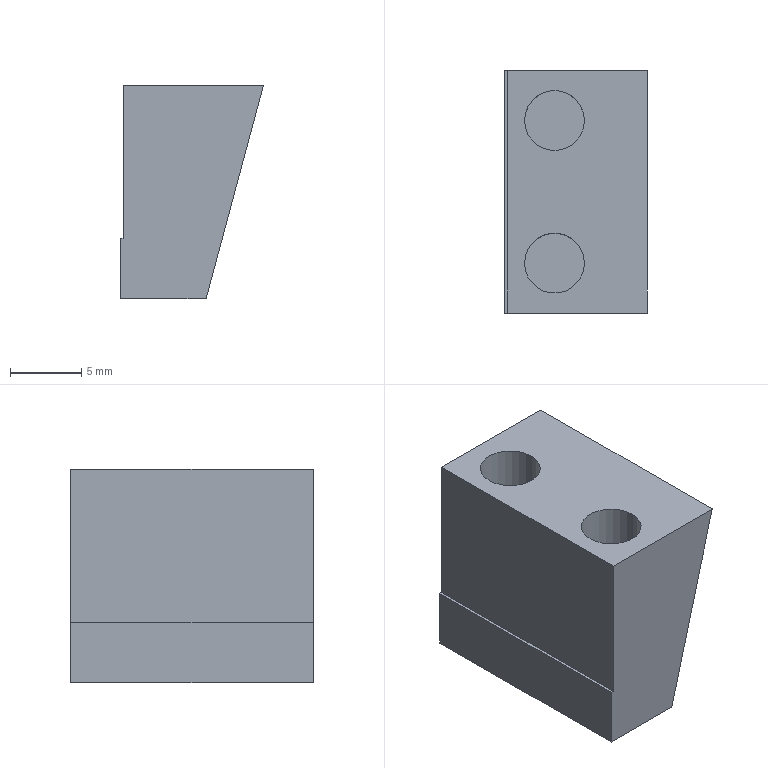Component | SolidWorks | 8TC-A15004-60-31A-4 | 1 solid | 14 faces | box 10.02 x 17 x 15 mm | volume 1770 mm3 | plane 10 | cylinder 4 | commonest cylinder face diameters 4.2 x4 | material #45
build123d program:
from build123d import *

# Parameters (mm, degrees)
BOSS_EXTRUDE1_DEPTH      = 8.5
M4_CLEARANCE_HOLE1_D     = 4.2
M4_CLEARANCE_HOLE1_DEPTH = 8.5
SKETCH1_W                = 0.7
SKETCH1_H                = 11.25
BLADESEATRELIEF_DEPTH    = 15


with BuildPart() as part:
    # Sketch1_2 → Boss-Extrude1 (new, symmetric)
    with BuildSketch(Plane(origin=(0, 0, 0), x_dir=(1, 0, 0), z_dir=(0, 1, 0))):
        Polygon((-7.019, 0), (3, 0), (3, 15), (-3, 15), align=None)
    extrude(amount=BOSS_EXTRUDE1_DEPTH, both=True)

    # M4 Clearance Hole1
    with Locations(Plane.XY):
        with Locations((-0.5, 5), (-0.5, -5)):
            Hole(M4_CLEARANCE_HOLE1_D / 2, depth=M4_CLEARANCE_HOLE1_DEPTH)

    # Sketch1 → BladeSeatRelief (cut, symmetric)
    with BuildSketch(Plane(origin=(0, 0, 0), x_dir=(1, 0, 0), z_dir=(0, 1, 0))):
        with Locations((3.15, 5.125)):
            Rectangle(SKETCH1_W, SKETCH1_H)
    extrude(amount=BLADESEATRELIEF_DEPTH, both=True, mode=Mode.SUBTRACT)


solid = part.part

# Placed as in the assembly
solid = solid.moved(Location((47.714, -68.5, 6), (0, 0, 180)))
STEP:
#1=COLOUR_RGB('',0.7922,0.8196,0.9333);
#2=FILL_AREA_STYLE_COLOUR('',#1);
#3=FILL_AREA_STYLE('',(#2));
#4=SURFACE_STYLE_FILL_AREA(#3);
#5=SURFACE_SIDE_STYLE('',(#4));
#6=SURFACE_STYLE_USAGE(.BOTH.,#5);
#7=PRESENTATION_STYLE_ASSIGNMENT((#6));
#8=CARTESIAN_POINT('',(1.981,-2.894,-0.09843));
#9=VERTEX_POINT('',#8);
#10=CARTESIAN_POINT('',(1.816,-2.894,-0.09843));
#11=VERTEX_POINT('',#10);
#12=CARTESIAN_POINT('',(1.898,-2.894,-0.09843));
#13=DIRECTION('',(0.,-0.,1.));
#14=DIRECTION('',(-1.,0.,0.));
#15=AXIS2_PLACEMENT_3D('',#12,#13,#14);
#16=CIRCLE('',#15,0.08268);
#17=EDGE_CURVE('',#9,#11,#16,.T.);
#18=ORIENTED_EDGE('',*,*,#17,.F.);
#19=CARTESIAN_POINT('',(1.981,-2.894,0.2362));
#20=VERTEX_POINT('',#19);
#21=CARTESIAN_POINT('',(1.981,-2.894,0.2362));
#22=DIRECTION('',(0.,-0.,1.));
#23=VECTOR('',#22,39.37);
#24=LINE('',#21,#23);
#25=EDGE_CURVE('',#9,#20,#24,.T.);
#26=ORIENTED_EDGE('',*,*,#25,.T.);
#27=CARTESIAN_POINT('',(1.816,-2.894,0.2362));
#28=VERTEX_POINT('',#27);
#29=CARTESIAN_POINT('',(1.898,-2.894,0.2362));
#30=DIRECTION('',(0.,-0.,1.));
#31=DIRECTION('',(-1.,0.,0.));
#32=AXIS2_PLACEMENT_3D('',#29,#30,#31);
#33=CIRCLE('',#32,0.08268);
#34=EDGE_CURVE('',#20,#28,#33,.T.);
#35=ORIENTED_EDGE('',*,*,#34,.T.);
#36=CARTESIAN_POINT('',(1.816,-2.894,0.2362));
#37=DIRECTION('',(0.,-0.,1.));
#38=VECTOR('',#37,39.37);
#39=LINE('',#36,#38);
#40=EDGE_CURVE('',#11,#28,#39,.T.);
#41=ORIENTED_EDGE('',*,*,#40,.F.);
#42=EDGE_LOOP('',(#18,#26,#35,#41));
#43=FACE_OUTER_BOUND('',#42,.T.);
#44=CARTESIAN_POINT('',(1.898,-2.894,0.2362));
#45=DIRECTION('',(0.,-0.,1.));
#46=DIRECTION('',(-1.,0.,0.));
#47=AXIS2_PLACEMENT_3D('',#44,#45,#46);
#48=CYLINDRICAL_SURFACE('',#47,0.08268);
#49=ADVANCED_FACE('',(#43),#48,.F.);
#50=CARTESIAN_POINT('',(1.981,-2.5,-0.09843));
#51=VERTEX_POINT('',#50);
#52=CARTESIAN_POINT('',(1.816,-2.5,-0.09843));
#53=VERTEX_POINT('',#52);
#54=CARTESIAN_POINT('',(1.898,-2.5,-0.09843));
#55=DIRECTION('',(0.,-0.,1.));
#56=DIRECTION('',(-1.,0.,0.));
#57=AXIS2_PLACEMENT_3D('',#54,#55,#56);
#58=CIRCLE('',#57,0.08268);
#59=EDGE_CURVE('',#51,#53,#58,.T.);
#60=ORIENTED_EDGE('',*,*,#59,.F.);
#61=CARTESIAN_POINT('',(1.981,-2.5,0.2362));
#62=VERTEX_POINT('',#61);
#63=CARTESIAN_POINT('',(1.981,-2.5,0.2362));
#64=DIRECTION('',(0.,-0.,1.));
#65=VECTOR('',#64,39.37);
#66=LINE('',#63,#65);
#67=EDGE_CURVE('',#51,#62,#66,.T.);
#68=ORIENTED_EDGE('',*,*,#67,.T.);
#69=CARTESIAN_POINT('',(1.816,-2.5,0.2362));
#70=VERTEX_POINT('',#69);
#71=CARTESIAN_POINT('',(1.898,-2.5,0.2362));
#72=DIRECTION('',(0.,-0.,1.));
#73=DIRECTION('',(-1.,0.,0.));
#74=AXIS2_PLACEMENT_3D('',#71,#72,#73);
#75=CIRCLE('',#74,0.08268);
#76=EDGE_CURVE('',#62,#70,#75,.T.);
#77=ORIENTED_EDGE('',*,*,#76,.T.);
#78=CARTESIAN_POINT('',(1.816,-2.5,0.2362));
#79=DIRECTION('',(0.,-0.,1.));
#80=VECTOR('',#79,39.37);
#81=LINE('',#78,#80);
#82=EDGE_CURVE('',#53,#70,#81,.T.);
#83=ORIENTED_EDGE('',*,*,#82,.F.);
#84=EDGE_LOOP('',(#60,#68,#77,#83));
#85=FACE_OUTER_BOUND('',#84,.T.);
#86=CARTESIAN_POINT('',(1.898,-2.5,0.2362));
#87=DIRECTION('',(0.,-0.,1.));
#88=DIRECTION('',(-1.,0.,0.));
#89=AXIS2_PLACEMENT_3D('',#86,#87,#88);
#90=CYLINDRICAL_SURFACE('',#89,0.08268);
#91=ADVANCED_FACE('',(#85),#90,.F.);
#92=CARTESIAN_POINT('',(1.76,-3.031,-0.187));
#93=VERTEX_POINT('',#92);
#94=CARTESIAN_POINT('',(1.76,-3.031,-0.3543));
#95=VERTEX_POINT('',#94);
#96=CARTESIAN_POINT('',(1.76,-3.031,0.2362));
#97=DIRECTION('',(-0.,0.,-1.));
#98=VECTOR('',#97,39.37);
#99=LINE('',#96,#98);
#100=EDGE_CURVE('',#93,#95,#99,.T.);
#101=ORIENTED_EDGE('',*,*,#100,.F.);
#102=CARTESIAN_POINT('',(1.76,-2.362,-0.187));
#103=VERTEX_POINT('',#102);
#104=CARTESIAN_POINT('',(1.76,-3.031,-0.187));
#105=DIRECTION('',(-0.,1.,0.));
#106=VECTOR('',#105,39.37);
#107=LINE('',#104,#106);
#108=EDGE_CURVE('',#93,#103,#107,.T.);
#109=ORIENTED_EDGE('',*,*,#108,.T.);
#110=CARTESIAN_POINT('',(1.76,-2.362,-0.3543));
#111=VERTEX_POINT('',#110);
#112=CARTESIAN_POINT('',(1.76,-2.362,0.2362));
#113=DIRECTION('',(-0.,0.,-1.));
#114=VECTOR('',#113,39.37);
#115=LINE('',#112,#114);
#116=EDGE_CURVE('',#103,#111,#115,.T.);
#117=ORIENTED_EDGE('',*,*,#116,.T.);
#118=CARTESIAN_POINT('',(1.76,-3.031,-0.3543));
#119=DIRECTION('',(-0.,1.,0.));
#120=VECTOR('',#119,39.37);
#121=LINE('',#118,#120);
#122=EDGE_CURVE('',#95,#111,#121,.T.);
#123=ORIENTED_EDGE('',*,*,#122,.F.);
#124=EDGE_LOOP('',(#101,#109,#117,#123));
#125=FACE_OUTER_BOUND('',#124,.T.);
#126=CARTESIAN_POINT('',(1.76,-3.031,0.2362));
#127=DIRECTION('',(1.,0.,-0.));
#128=DIRECTION('',(0.,-0.,1.));
#129=AXIS2_PLACEMENT_3D('',#126,#127,#128);
#130=PLANE('',#129);
#131=ADVANCED_FACE('',(#125),#130,.F.);
#132=CARTESIAN_POINT('',(1.997,-2.362,-0.3543));
#133=VERTEX_POINT('',#132);
#134=CARTESIAN_POINT('',(1.76,-2.362,-0.3543));
#135=DIRECTION('',(1.,0.,-0.));
#136=VECTOR('',#135,39.37);
#137=LINE('',#134,#136);
#138=EDGE_CURVE('',#111,#133,#137,.T.);
#139=ORIENTED_EDGE('',*,*,#138,.T.);
#140=CARTESIAN_POINT('',(1.997,-3.031,-0.3543));
#141=VERTEX_POINT('',#140);
#142=CARTESIAN_POINT('',(1.997,-3.031,-0.3543));
#143=DIRECTION('',(-0.,1.,0.));
#144=VECTOR('',#143,39.37);
#145=LINE('',#142,#144);
#146=EDGE_CURVE('',#141,#133,#145,.T.);
#147=ORIENTED_EDGE('',*,*,#146,.F.);
#148=CARTESIAN_POINT('',(1.76,-3.031,-0.3543));
#149=DIRECTION('',(1.,0.,-0.));
#150=VECTOR('',#149,39.37);
#151=LINE('',#148,#150);
#152=EDGE_CURVE('',#95,#141,#151,.T.);
#153=ORIENTED_EDGE('',*,*,#152,.F.);
#154=ORIENTED_EDGE('',*,*,#122,.T.);
#155=EDGE_LOOP('',(#139,#147,#153,#154));
#156=FACE_OUTER_BOUND('',#155,.T.);
#157=CARTESIAN_POINT('',(1.76,-3.031,-0.3543));
#158=DIRECTION('',(0.,-0.,1.));
#159=DIRECTION('',(-1.,-0.,0.));
#160=AXIS2_PLACEMENT_3D('',#157,#158,#159);
#161=PLANE('',#160);
#162=ADVANCED_FACE('',(#156),#161,.F.);
#163=CARTESIAN_POINT('',(2.155,-2.362,0.2362));
#164=VERTEX_POINT('',#163);
#165=CARTESIAN_POINT('',(2.155,-2.362,0.2362));
#166=DIRECTION('',(0.2588,-0.,0.9659));
#167=VECTOR('',#166,39.37);
#168=LINE('',#165,#167);
#169=EDGE_CURVE('',#133,#164,#168,.T.);
#170=ORIENTED_EDGE('',*,*,#169,.T.);
#171=CARTESIAN_POINT('',(2.155,-3.031,0.2362));
#172=VERTEX_POINT('',#171);
#173=CARTESIAN_POINT('',(2.155,-3.031,0.2362));
#174=DIRECTION('',(-0.,1.,0.));
#175=VECTOR('',#174,39.37);
#176=LINE('',#173,#175);
#177=EDGE_CURVE('',#172,#164,#176,.T.);
#178=ORIENTED_EDGE('',*,*,#177,.F.);
#179=CARTESIAN_POINT('',(2.155,-3.031,0.2362));
#180=DIRECTION('',(0.2588,-0.,0.9659));
#181=VECTOR('',#180,39.37);
#182=LINE('',#179,#181);
#183=EDGE_CURVE('',#141,#172,#182,.T.);
#184=ORIENTED_EDGE('',*,*,#183,.F.);
#185=ORIENTED_EDGE('',*,*,#146,.T.);
#186=EDGE_LOOP('',(#170,#178,#184,#185));
#187=FACE_OUTER_BOUND('',#186,.T.);
#188=CARTESIAN_POINT('',(2.155,-3.031,0.2362));
#189=DIRECTION('',(-0.9659,-0.,0.2588));
#190=DIRECTION('',(-0.2588,0.,-0.9659));
#191=AXIS2_PLACEMENT_3D('',#188,#189,#190);
#192=PLANE('',#191);
#193=ADVANCED_FACE('',(#187),#192,.F.);
#194=CARTESIAN_POINT('',(1.898,-2.894,0.2362));
#195=DIRECTION('',(0.,-0.,1.));
#196=DIRECTION('',(-1.,0.,0.));
#197=AXIS2_PLACEMENT_3D('',#194,#195,#196);
#198=CIRCLE('',#197,0.08268);
#199=EDGE_CURVE('',#28,#20,#198,.T.);
#200=ORIENTED_EDGE('',*,*,#199,.F.);
#201=ORIENTED_EDGE('',*,*,#34,.F.);
#202=EDGE_LOOP('',(#200,#201));
#203=FACE_BOUND('',#202,.T.);
#204=CARTESIAN_POINT('',(1.898,-2.5,0.2362));
#205=DIRECTION('',(0.,-0.,1.));
#206=DIRECTION('',(-1.,0.,0.));
#207=AXIS2_PLACEMENT_3D('',#204,#205,#206);
#208=CIRCLE('',#207,0.08268);
#209=EDGE_CURVE('',#70,#62,#208,.T.);
#210=ORIENTED_EDGE('',*,*,#209,.F.);
#211=ORIENTED_EDGE('',*,*,#76,.F.);
#212=EDGE_LOOP('',(#210,#211));
#213=FACE_BOUND('',#212,.T.);
#214=CARTESIAN_POINT('',(1.768,-2.362,0.2362));
#215=VERTEX_POINT('',#214);
#216=CARTESIAN_POINT('',(2.155,-2.362,0.2362));
#217=DIRECTION('',(-1.,-0.,0.));
#218=VECTOR('',#217,39.37);
#219=LINE('',#216,#218);
#220=EDGE_CURVE('',#164,#215,#219,.T.);
#221=ORIENTED_EDGE('',*,*,#220,.T.);
#222=CARTESIAN_POINT('',(1.768,-3.031,0.2362));
#223=VERTEX_POINT('',#222);
#224=CARTESIAN_POINT('',(1.768,-3.031,0.2362));
#225=DIRECTION('',(0.,-1.,-0.));
#226=VECTOR('',#225,39.37);
#227=LINE('',#224,#226);
#228=EDGE_CURVE('',#215,#223,#227,.T.);
#229=ORIENTED_EDGE('',*,*,#228,.T.);
#230=CARTESIAN_POINT('',(2.155,-3.031,0.2362));
#231=DIRECTION('',(-1.,-0.,0.));
#232=VECTOR('',#231,39.37);
#233=LINE('',#230,#232);
#234=EDGE_CURVE('',#172,#223,#233,.T.);
#235=ORIENTED_EDGE('',*,*,#234,.F.);
#236=ORIENTED_EDGE('',*,*,#177,.T.);
#237=EDGE_LOOP('',(#221,#229,#235,#236));
#238=FACE_OUTER_BOUND('',#237,.T.);
#239=CARTESIAN_POINT('',(2.155,-3.031,0.2362));
#240=DIRECTION('',(-0.,0.,-1.));
#241=DIRECTION('',(1.,0.,-0.));
#242=AXIS2_PLACEMENT_3D('',#239,#240,#241);
#243=PLANE('',#242);
#244=ADVANCED_FACE('',(#203,#213,#238),#243,.F.);
#245=CARTESIAN_POINT('',(1.768,-3.031,-0.187));
#246=VERTEX_POINT('',#245);
#247=CARTESIAN_POINT('',(1.768,-3.031,0.2362));
#248=DIRECTION('',(0.,-0.,1.));
#249=VECTOR('',#248,39.37);
#250=LINE('',#247,#249);
#251=EDGE_CURVE('',#246,#223,#250,.T.);
#252=ORIENTED_EDGE('',*,*,#251,.F.);
#253=CARTESIAN_POINT('',(1.879,-3.031,-0.187));
#254=DIRECTION('',(1.,0.,-0.));
#255=VECTOR('',#254,39.37);
#256=LINE('',#253,#255);
#257=EDGE_CURVE('',#93,#246,#256,.T.);
#258=ORIENTED_EDGE('',*,*,#257,.F.);
#259=ORIENTED_EDGE('',*,*,#100,.T.);
#260=ORIENTED_EDGE('',*,*,#152,.T.);
#261=ORIENTED_EDGE('',*,*,#183,.T.);
#262=ORIENTED_EDGE('',*,*,#234,.T.);
#263=EDGE_LOOP('',(#252,#258,#259,#260,#261,#262));
#264=FACE_OUTER_BOUND('',#263,.T.);
#265=CARTESIAN_POINT('',(1.879,-3.031,0.2362));
#266=DIRECTION('',(0.,-1.,-0.));
#267=DIRECTION('',(0.,-0.,1.));
#268=AXIS2_PLACEMENT_3D('',#265,#266,#267);
#269=PLANE('',#268);
#270=ADVANCED_FACE('',(#264),#269,.T.);
#271=CARTESIAN_POINT('',(1.768,-2.362,-0.187));
#272=VERTEX_POINT('',#271);
#273=CARTESIAN_POINT('',(1.879,-2.362,-0.187));
#274=DIRECTION('',(1.,0.,-0.));
#275=VECTOR('',#274,39.37);
#276=LINE('',#273,#275);
#277=EDGE_CURVE('',#103,#272,#276,.T.);
#278=ORIENTED_EDGE('',*,*,#277,.T.);
#279=CARTESIAN_POINT('',(1.768,-2.362,0.2362));
#280=DIRECTION('',(0.,-0.,1.));
#281=VECTOR('',#280,39.37);
#282=LINE('',#279,#281);
#283=EDGE_CURVE('',#272,#215,#282,.T.);
#284=ORIENTED_EDGE('',*,*,#283,.T.);
#285=ORIENTED_EDGE('',*,*,#220,.F.);
#286=ORIENTED_EDGE('',*,*,#169,.F.);
#287=ORIENTED_EDGE('',*,*,#138,.F.);
#288=ORIENTED_EDGE('',*,*,#116,.F.);
#289=EDGE_LOOP('',(#278,#284,#285,#286,#287,#288));
#290=FACE_OUTER_BOUND('',#289,.T.);
#291=CARTESIAN_POINT('',(1.879,-2.362,0.2362));
#292=DIRECTION('',(0.,-1.,-0.));
#293=DIRECTION('',(0.,-0.,1.));
#294=AXIS2_PLACEMENT_3D('',#291,#292,#293);
#295=PLANE('',#294);
#296=ADVANCED_FACE('',(#290),#295,.F.);
#297=CARTESIAN_POINT('',(1.898,-2.5,-0.09843));
#298=DIRECTION('',(0.,-0.,1.));
#299=DIRECTION('',(-1.,0.,0.));
#300=AXIS2_PLACEMENT_3D('',#297,#298,#299);
#301=CIRCLE('',#300,0.08268);
#302=EDGE_CURVE('',#53,#51,#301,.T.);
#303=ORIENTED_EDGE('',*,*,#302,.T.);
#304=ORIENTED_EDGE('',*,*,#59,.T.);
#305=EDGE_LOOP('',(#303,#304));
#306=FACE_OUTER_BOUND('',#305,.T.);
#307=CARTESIAN_POINT('',(1.898,-2.5,-0.09843));
#308=DIRECTION('',(-0.,0.,-1.));
#309=DIRECTION('',(1.,0.,-0.));
#310=AXIS2_PLACEMENT_3D('',#307,#308,#309);
#311=PLANE('',#310);
#312=ADVANCED_FACE('',(#306),#311,.F.);
#313=ORIENTED_EDGE('',*,*,#67,.F.);
#314=ORIENTED_EDGE('',*,*,#302,.F.);
#315=ORIENTED_EDGE('',*,*,#82,.T.);
#316=ORIENTED_EDGE('',*,*,#209,.T.);
#317=EDGE_LOOP('',(#313,#314,#315,#316));
#318=FACE_OUTER_BOUND('',#317,.T.);
#319=CARTESIAN_POINT('',(1.898,-2.5,0.2362));
#320=DIRECTION('',(0.,-0.,1.));
#321=DIRECTION('',(-1.,0.,0.));
#322=AXIS2_PLACEMENT_3D('',#319,#320,#321);
#323=CYLINDRICAL_SURFACE('',#322,0.08268);
#324=ADVANCED_FACE('',(#318),#323,.F.);
#325=CARTESIAN_POINT('',(1.898,-2.894,-0.09843));
#326=DIRECTION('',(0.,-0.,1.));
#327=DIRECTION('',(-1.,0.,0.));
#328=AXIS2_PLACEMENT_3D('',#325,#326,#327);
#329=CIRCLE('',#328,0.08268);
#330=EDGE_CURVE('',#11,#9,#329,.T.);
#331=ORIENTED_EDGE('',*,*,#330,.T.);
#332=ORIENTED_EDGE('',*,*,#17,.T.);
#333=EDGE_LOOP('',(#331,#332));
#334=FACE_OUTER_BOUND('',#333,.T.);
#335=CARTESIAN_POINT('',(1.898,-2.894,-0.09843));
#336=DIRECTION('',(-0.,0.,-1.));
#337=DIRECTION('',(1.,0.,-0.));
#338=AXIS2_PLACEMENT_3D('',#335,#336,#337);
#339=PLANE('',#338);
#340=ADVANCED_FACE('',(#334),#339,.F.);
#341=ORIENTED_EDGE('',*,*,#25,.F.);
#342=ORIENTED_EDGE('',*,*,#330,.F.);
#343=ORIENTED_EDGE('',*,*,#40,.T.);
#344=ORIENTED_EDGE('',*,*,#199,.T.);
#345=EDGE_LOOP('',(#341,#342,#343,#344));
#346=FACE_OUTER_BOUND('',#345,.T.);
#347=CARTESIAN_POINT('',(1.898,-2.894,0.2362));
#348=DIRECTION('',(0.,-0.,1.));
#349=DIRECTION('',(-1.,0.,0.));
#350=AXIS2_PLACEMENT_3D('',#347,#348,#349);
#351=CYLINDRICAL_SURFACE('',#350,0.08268);
#352=ADVANCED_FACE('',(#346),#351,.F.);
#353=ORIENTED_EDGE('',*,*,#251,.T.);
#354=ORIENTED_EDGE('',*,*,#228,.F.);
#355=ORIENTED_EDGE('',*,*,#283,.F.);
#356=CARTESIAN_POINT('',(1.768,-2.106,-0.187));
#357=DIRECTION('',(0.,-1.,-0.));
#358=VECTOR('',#357,39.37);
#359=LINE('',#356,#358);
#360=EDGE_CURVE('',#272,#246,#359,.T.);
#361=ORIENTED_EDGE('',*,*,#360,.T.);
#362=EDGE_LOOP('',(#353,#354,#355,#361));
#363=FACE_OUTER_BOUND('',#362,.T.);
#364=CARTESIAN_POINT('',(1.768,-2.106,-0.187));
#365=DIRECTION('',(1.,0.,-0.));
#366=DIRECTION('',(0.,-0.,1.));
#367=AXIS2_PLACEMENT_3D('',#364,#365,#366);
#368=PLANE('',#367);
#369=ADVANCED_FACE('',(#363),#368,.F.);
#370=ORIENTED_EDGE('',*,*,#257,.T.);
#371=ORIENTED_EDGE('',*,*,#360,.F.);
#372=ORIENTED_EDGE('',*,*,#277,.F.);
#373=ORIENTED_EDGE('',*,*,#108,.F.);
#374=EDGE_LOOP('',(#370,#371,#372,#373));
#375=FACE_OUTER_BOUND('',#374,.T.);
#376=CARTESIAN_POINT('',(1.768,-2.106,-0.187));
#377=DIRECTION('',(-0.,0.,-1.));
#378=DIRECTION('',(1.,0.,-0.));
#379=AXIS2_PLACEMENT_3D('',#376,#377,#378);
#380=PLANE('',#379);
#381=ADVANCED_FACE('',(#375),#380,.F.);
#382=CLOSED_SHELL('',(#49,#91,#131,#162,#193,#244,#270,#296,#312,#324,#340,#352,#369,#381));
#383=MANIFOLD_SOLID_BREP('',#382);
#384=STYLED_ITEM('',(#7),#383);
#385=(LENGTH_UNIT()NAMED_UNIT(*)SI_UNIT($,.METRE.));
#386=LENGTH_MEASURE_WITH_UNIT(LENGTH_MEASURE(0.0254),#385);
#387=DIMENSIONAL_EXPONENTS(1.,0.,0.,0.,0.,0.,0.);
#388=(CONVERSION_BASED_UNIT('',#386)LENGTH_UNIT()NAMED_UNIT(#387));
#389=UNCERTAINTY_MEASURE_WITH_UNIT(LENGTH_MEASURE(0.00001),#388,'','');
#390=(NAMED_UNIT(*)PLANE_ANGLE_UNIT()SI_UNIT($,.RADIAN.));
#391=(NAMED_UNIT(*)SI_UNIT($,.STERADIAN.)SOLID_ANGLE_UNIT());
#392=(GEOMETRIC_REPRESENTATION_CONTEXT(3)GLOBAL_UNCERTAINTY_ASSIGNED_CONTEXT((#389))GLOBAL_UNIT_ASSIGNED_CONTEXT((#388,#390,#391))REPRESENTATION_CONTEXT('',''));
#393=MECHANICAL_DESIGN_GEOMETRIC_PRESENTATION_REPRESENTATION('',(#384),#392);
#394=PRESENTATION_LAYER_ASSIGNMENT('','',(#384));
#395=CARTESIAN_POINT('',(0.,0.,0.));
#396=DIRECTION('',(0.,0.,1.));
#397=DIRECTION('',(1.,0.,0.));
#398=AXIS2_PLACEMENT_3D('',#395,#396,#397);
#399=(LENGTH_UNIT()NAMED_UNIT(*)SI_UNIT($,.METRE.));
#400=LENGTH_MEASURE_WITH_UNIT(LENGTH_MEASURE(0.0254),#399);
#401=DIMENSIONAL_EXPONENTS(1.,0.,0.,0.,0.,0.,0.);
#402=(CONVERSION_BASED_UNIT('',#400)LENGTH_UNIT()NAMED_UNIT(#401));
#403=UNCERTAINTY_MEASURE_WITH_UNIT(LENGTH_MEASURE(0.00001),#402,'','');
#404=(NAMED_UNIT(*)PLANE_ANGLE_UNIT()SI_UNIT($,.RADIAN.));
#405=(NAMED_UNIT(*)SI_UNIT($,.STERADIAN.)SOLID_ANGLE_UNIT());
#406=(GEOMETRIC_REPRESENTATION_CONTEXT(3)GLOBAL_UNCERTAINTY_ASSIGNED_CONTEXT((#403))GLOBAL_UNIT_ASSIGNED_CONTEXT((#402,#404,#405))REPRESENTATION_CONTEXT('',''));
#407=ADVANCED_BREP_SHAPE_REPRESENTATION('',(#383,#398),#406);